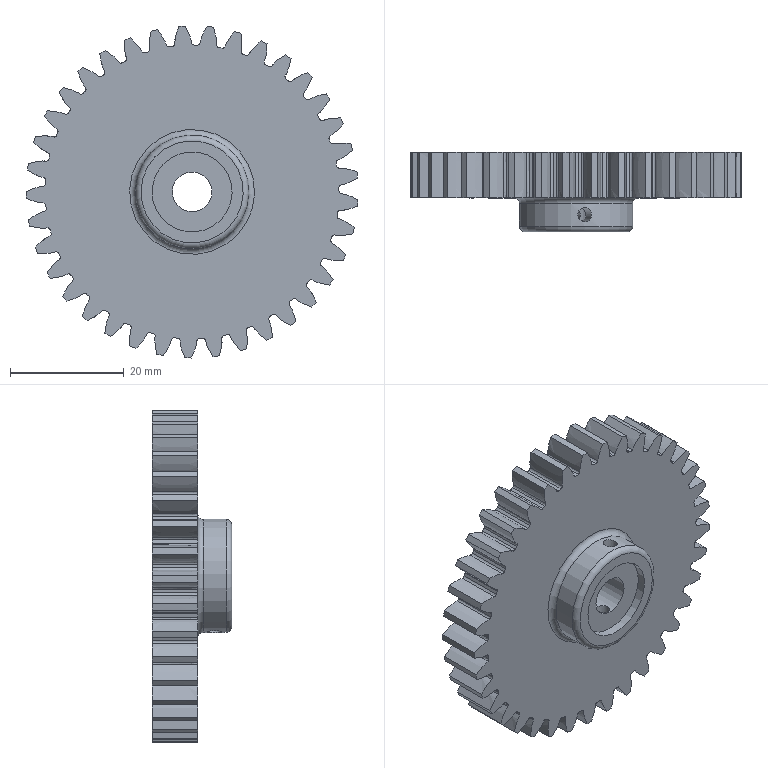Component | NX | LARGE_GEAR | 1 solid | 233 faces | volume 20286 mm3 | other 185 | cylinder 42 | plane 4 | torus 2 | commonest cylinder face diameters 51.75 x37 2.5 x2 20 x1 7 x1 14.1 x1